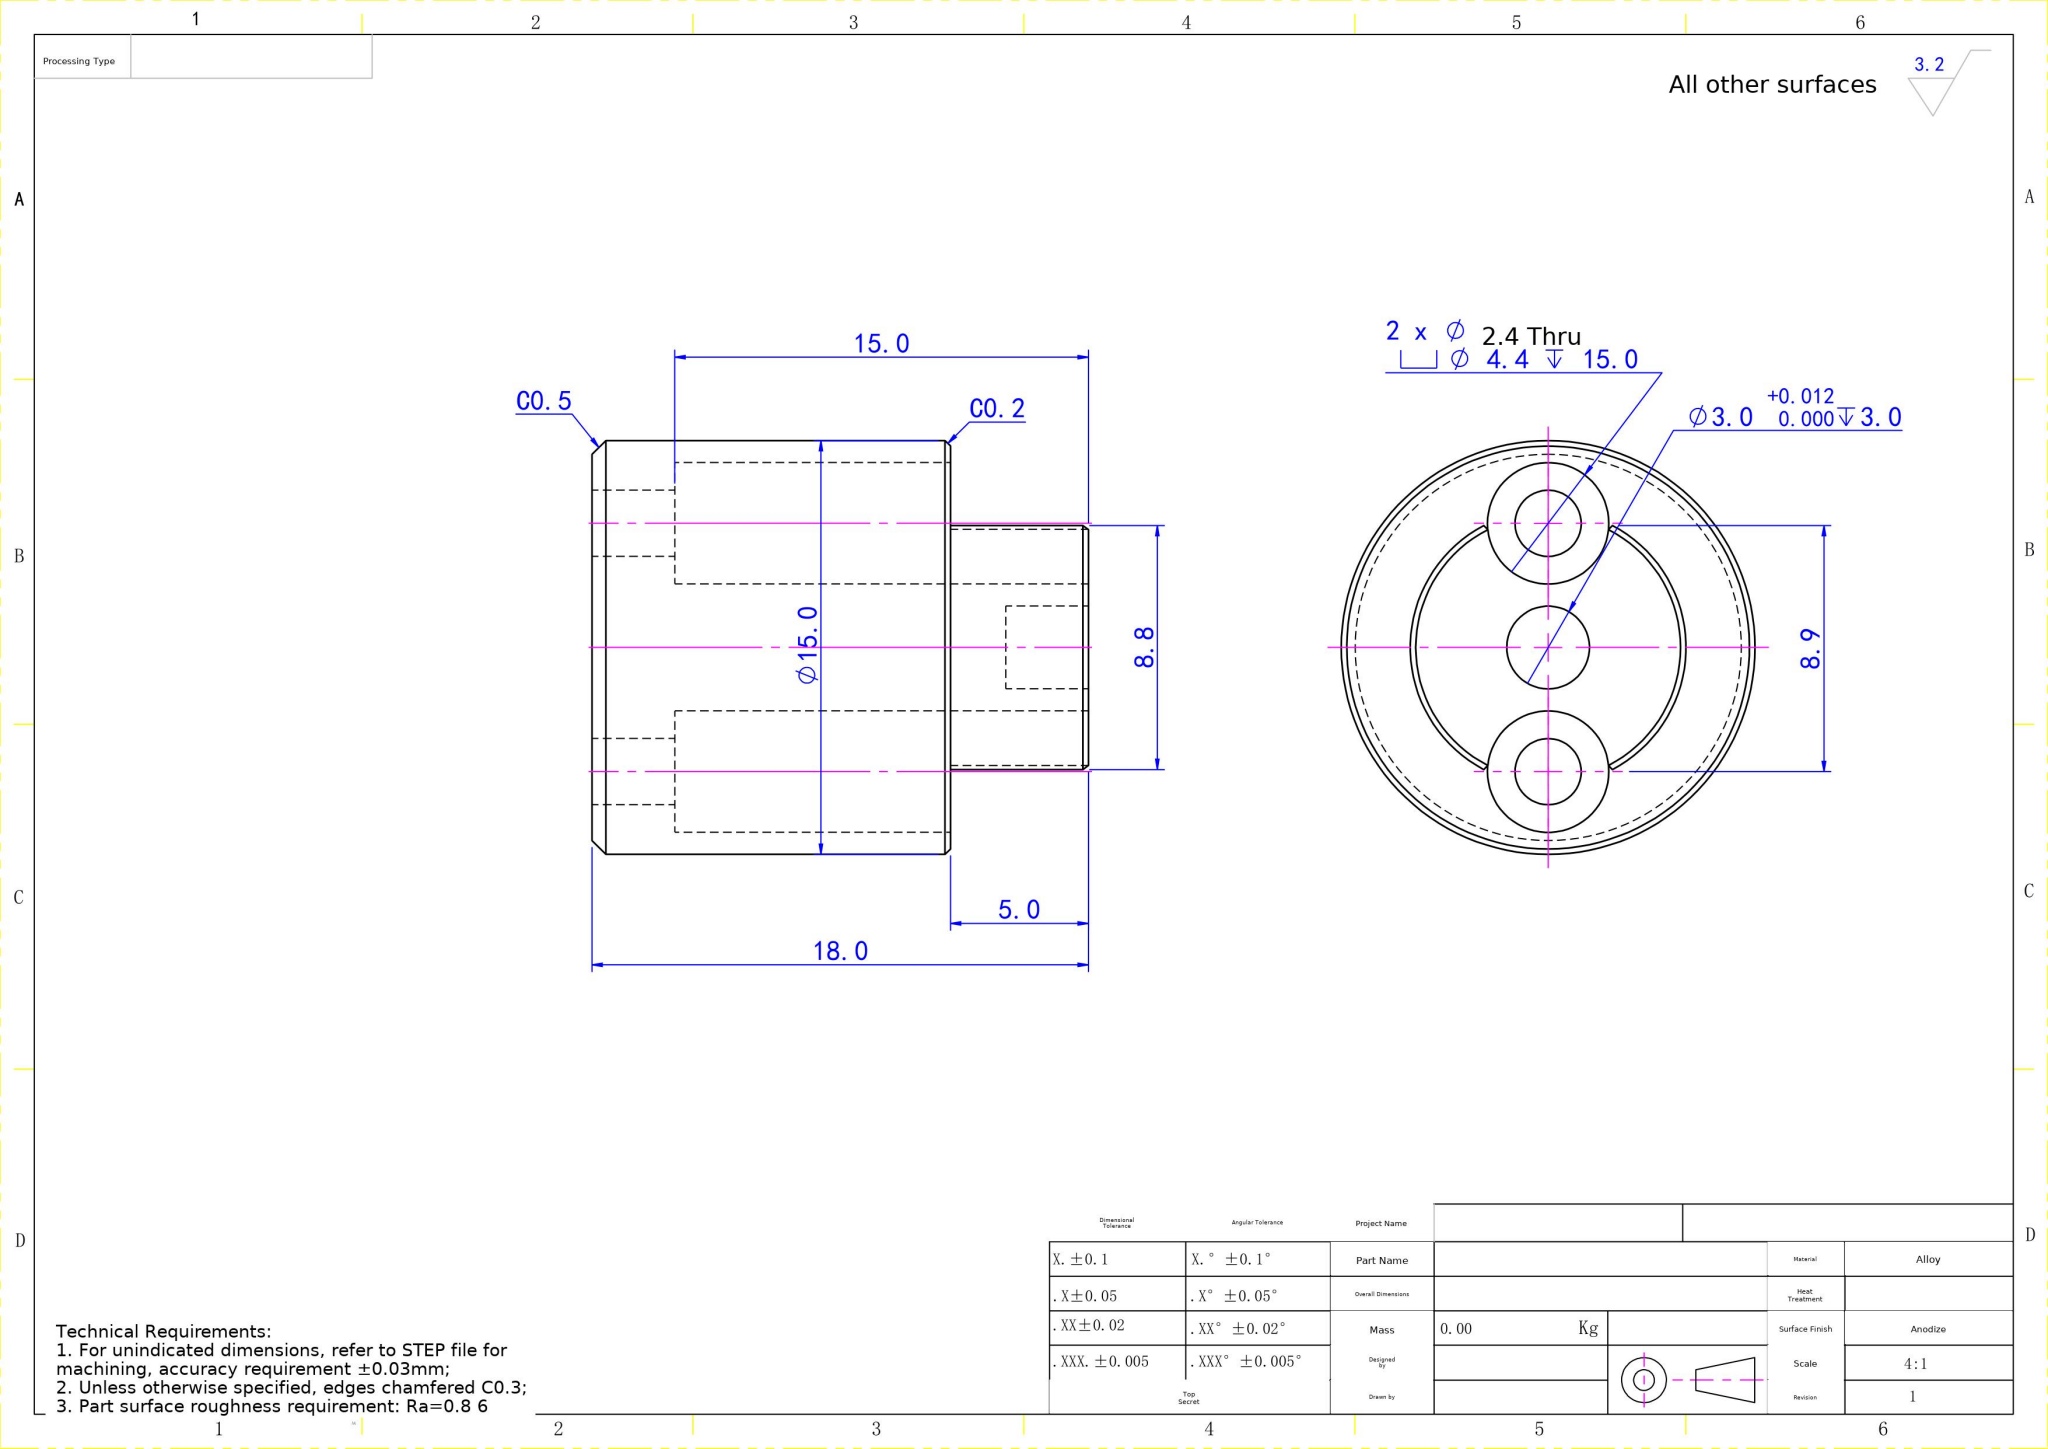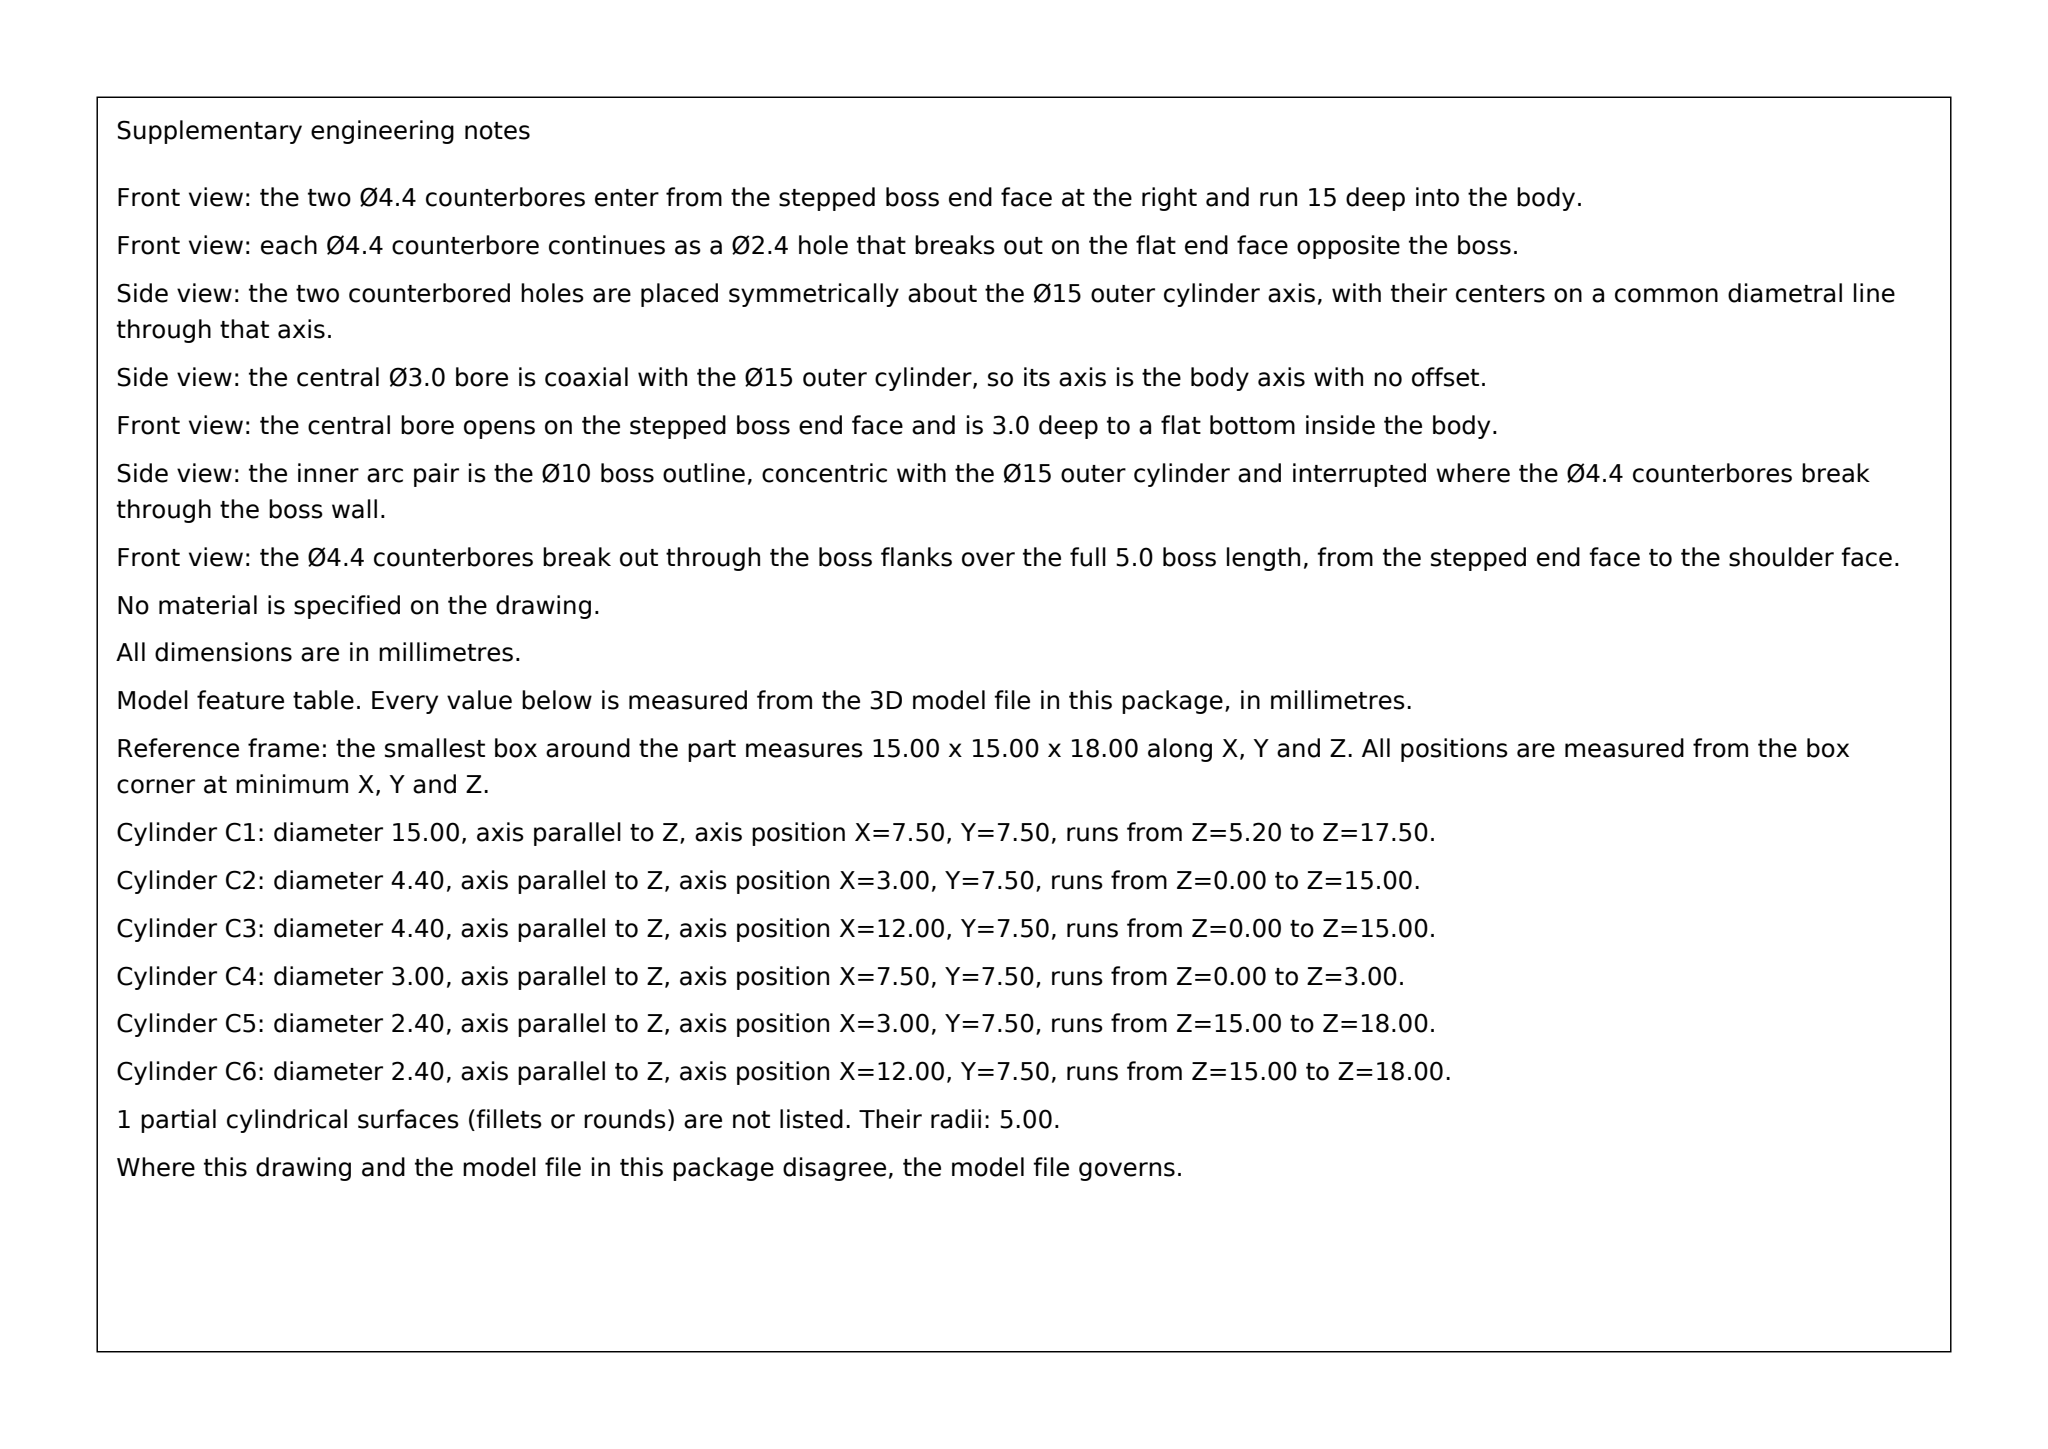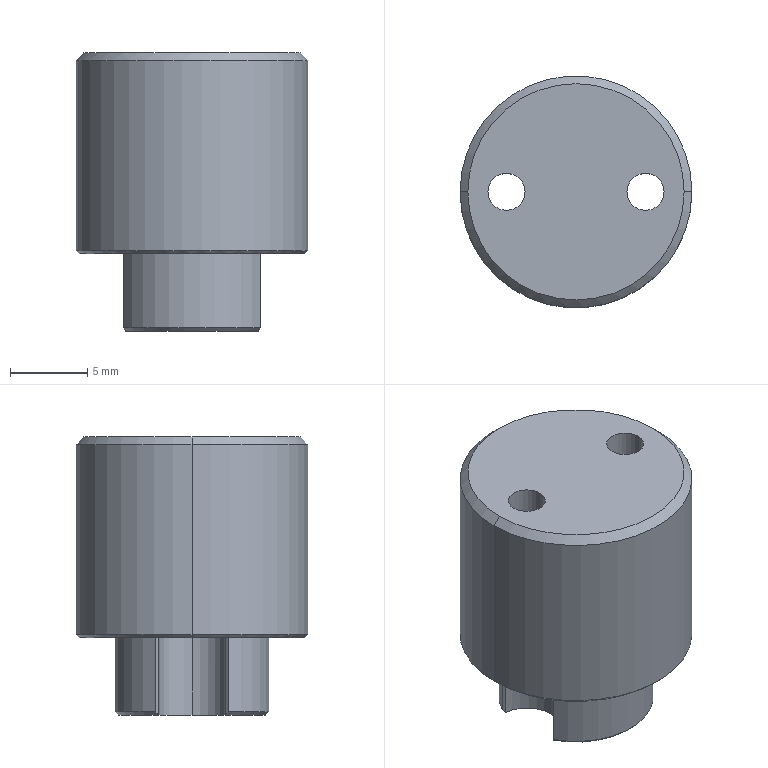Part | SolidWorks | mm | 1 solid | 30 faces | box 15 x 15 x 18 mm | volume 2239 mm3 | cylinder 14 | plane 10 | cone 6 | commonest cylinder face diameters 2.4 x4 4.4 x4 3 x2 15 x2 10 x2
Drawing notes:
C0.2 CHAMFER ON Ø10 BOSS END FACE | from the solid: cone 90° incl, ref dia 9.6 on Ø10 boss (10.0 cyl, len 4.8) => (10-9.6)/2 = 0.2 x 45°